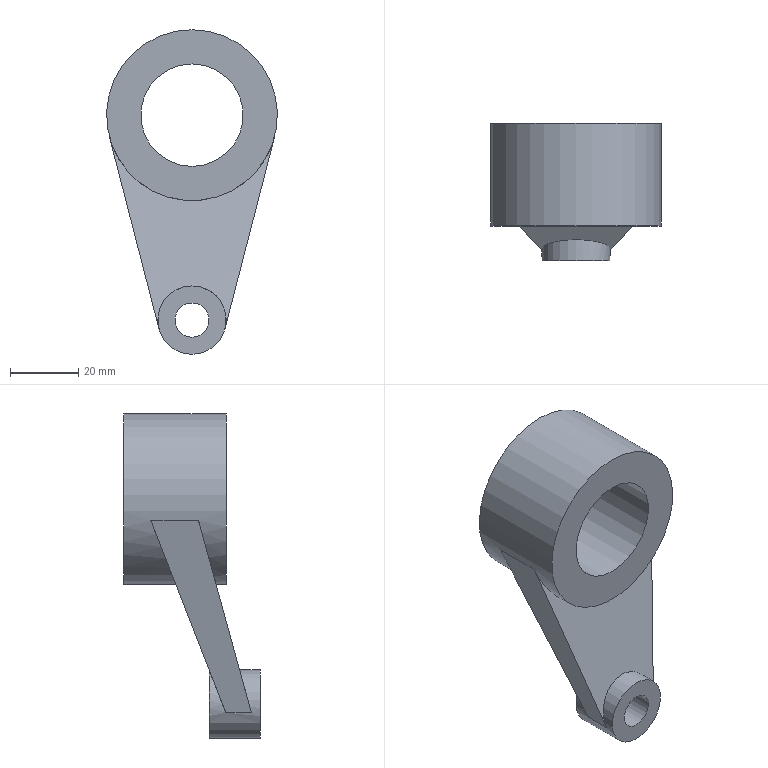Component | NX | WORKPIECE | 1 solid | 12 faces | box 50 x 40 x 95 mm | volume 52074 mm3 | plane 8 | cylinder 4 | commonest cylinder face diameters 50 x1 30 x1 20 x1 10 x1
STEP:
#1=CARTESIAN_POINT('',(0.,0.,0.));
#2=DIRECTION('',(0.,0.,1.));
#3=DIRECTION('',(1.,0.,0.));
#4=AXIS2_PLACEMENT_3D('',#1,#2,#3);
#5=CARTESIAN_POINT('',(-38.364,45.603,0.0009287));
#6=VERTEX_POINT('',#5);
#7=CARTESIAN_POINT('',(-28.68,50.48,12.5));
#8=VERTEX_POINT('',#7);
#9=CARTESIAN_POINT('',(-28.681,46.579,2.5));
#10=DIRECTION('',(-0.00003485,0.9316,-0.3634));
#11=DIRECTION('',(-0.00008933,-0.3634,-0.9316));
#12=AXIS2_PLACEMENT_3D('',#9,#10,#11);
#13=ELLIPSE('',#12,10.734,10.);
#14=CARTESIAN_POINT('',(1.318,43.947,-4.249));
#15=DIRECTION('',(0.00003485,-0.9316,0.3634));
#16=DIRECTION('',(-0.00008933,-0.3634,-0.9316));
#17=AXIS2_PLACEMENT_3D('',#14,#15,#16);
#18=PLANE('',#17);
#19=CARTESIAN_POINT('',(3.492,-30.));
#20=CARTESIAN_POINT('',(3.492,-47.321));
#21=CARTESIAN_POINT('',(-12.609,-38.66));
#22=CARTESIAN_POINT('',(-28.71,-30.));
#23=CARTESIAN_POINT('',(-12.609,-21.34));
#24=CARTESIAN_POINT('',(3.492,-12.679));
#25=CARTESIAN_POINT('',(3.492,-30.));
#26=(BOUNDED_CURVE()B_SPLINE_CURVE(2,(#19,#20,#21,#22,#23,#24,#25),.UNSPECIFIED.,.T.,.F.)B_SPLINE_CURVE_WITH_KNOTS((1,2,2,2,2,1),(-2.094,0.,2.094,4.189,6.283,8.378),.UNSPECIFIED.)CURVE()GEOMETRIC_REPRESENTATION_ITEM()RATIONAL_B_SPLINE_CURVE((1.,0.5,1.,0.5,1.,0.5,1.))REPRESENTATION_ITEM(''));
#27=(GEOMETRIC_REPRESENTATION_CONTEXT(2)PARAMETRIC_REPRESENTATION_CONTEXT()REPRESENTATION_CONTEXT('',''));
#28=DEFINITIONAL_REPRESENTATION('',(#26),#27);
#29=PCURVE('',#18,#28);
#30=CARTESIAN_POINT('',(-28.681,50.5,2.5));
#31=DIRECTION('',(0.,-1.,0.));
#32=DIRECTION('',(-0.00009588,0.,-1.));
#33=AXIS2_PLACEMENT_3D('',#30,#31,#32);
#34=CYLINDRICAL_SURFACE('',#33,10.);
#35=CARTESIAN_POINT('',(4.965,4.897));
#36=CARTESIAN_POINT('',(4.91,4.688));
#37=CARTESIAN_POINT('',(4.799,4.261));
#38=CARTESIAN_POINT('',(4.634,3.613));
#39=CARTESIAN_POINT('',(4.468,2.972));
#40=CARTESIAN_POINT('',(4.302,2.358));
#41=CARTESIAN_POINT('',(4.136,1.786));
#42=CARTESIAN_POINT('',(3.97,1.273));
#43=CARTESIAN_POINT('',(3.805,0.8326));
#44=CARTESIAN_POINT('',(3.639,0.4769));
#45=CARTESIAN_POINT('',(3.473,0.2156));
#46=CARTESIAN_POINT('',(3.307,0.05589));
#47=CARTESIAN_POINT('',(3.142,0.002165));
#48=CARTESIAN_POINT('',(2.976,0.05589));
#49=CARTESIAN_POINT('',(2.81,0.2156));
#50=CARTESIAN_POINT('',(2.644,0.4769));
#51=CARTESIAN_POINT('',(2.479,0.8326));
#52=CARTESIAN_POINT('',(2.313,1.273));
#53=CARTESIAN_POINT('',(2.147,1.786));
#54=CARTESIAN_POINT('',(1.981,2.358));
#55=CARTESIAN_POINT('',(1.815,2.972));
#56=CARTESIAN_POINT('',(1.65,3.613));
#57=CARTESIAN_POINT('',(1.484,4.261));
#58=CARTESIAN_POINT('',(1.373,4.688));
#59=CARTESIAN_POINT('',(1.318,4.897));
#60=B_SPLINE_CURVE_WITH_KNOTS('',3,(#35,#36,#37,#38,#39,#40,#41,#42,#43,#44,#45,#46,#47,#48,#49,#50,#51,#52,#53,#54,#55,#56,#57,#58,#59),.UNSPECIFIED.,.F.,.F.,(4,1,1,1,1,1,1,1,1,1,1,1,1,1,1,1,1,1,1,1,1,1,4),(1.318,1.484,1.65,1.815,1.981,2.147,2.313,2.479,2.644,2.81,2.976,3.142,3.307,3.473,3.639,3.805,3.97,4.136,4.302,4.468,4.634,4.799,4.965),.QUASI_UNIFORM_KNOTS.);
#61=(GEOMETRIC_REPRESENTATION_CONTEXT(2)PARAMETRIC_REPRESENTATION_CONTEXT()REPRESENTATION_CONTEXT('',''));
#62=DEFINITIONAL_REPRESENTATION('',(#60),#61);
#63=PCURVE('',#34,#62);
#64=SURFACE_CURVE('',#13,(#29,#63),.PCURVE_S1.);
#65=EDGE_CURVE('',#6,#8,#64,.T.);
#66=ORIENTED_EDGE('',*,*,#65,.F.);
#67=CARTESIAN_POINT('',(-52.882,67.548,56.252));
#68=VERTEX_POINT('',#67);
#69=CARTESIAN_POINT('',(-35.158,40.758,-12.42));
#70=DIRECTION('',(-0.2338,0.3534,0.9058));
#71=VECTOR('',#70,1.);
#72=LINE('',#69,#71);
#73=CARTESIAN_POINT('',(8.774,-36.475));
#74=DIRECTION('',(-0.9723,-0.2339));
#75=VECTOR('',#74,1.);
#76=LINE('',#73,#75);
#77=(GEOMETRIC_REPRESENTATION_CONTEXT(2)PARAMETRIC_REPRESENTATION_CONTEXT()REPRESENTATION_CONTEXT('',''));
#78=DEFINITIONAL_REPRESENTATION('',(#76),#77);
#79=PCURVE('',#18,#78);
#80=CARTESIAN_POINT('',(-64.414,-24.5,100.934));
#81=DIRECTION('',(0.9683,0.,0.2499));
#82=DIRECTION('',(0.2499,0.,-0.9683));
#83=AXIS2_PLACEMENT_3D('',#80,#81,#82);
#84=PLANE('',#83);
#85=CARTESIAN_POINT('',(117.069,65.258));
#86=DIRECTION('',(-0.9355,0.3534));
#87=VECTOR('',#86,1.);
#88=LINE('',#85,#87);
#89=(GEOMETRIC_REPRESENTATION_CONTEXT(2)PARAMETRIC_REPRESENTATION_CONTEXT()REPRESENTATION_CONTEXT('',''));
#90=DEFINITIONAL_REPRESENTATION('',(#88),#89);
#91=PCURVE('',#84,#90);
#92=SURFACE_CURVE('',#72,(#79,#91),.PCURVE_S1.);
#93=EDGE_CURVE('',#6,#68,#92,.T.);
#94=ORIENTED_EDGE('',*,*,#93,.T.);
#95=CARTESIAN_POINT('',(-4.47,67.548,56.248));
#96=VERTEX_POINT('',#95);
#97=CARTESIAN_POINT('',(-28.675,69.986,62.5));
#98=DIRECTION('',(0.00003485,-0.9316,0.3634));
#99=DIRECTION('',(-0.00008933,-0.3634,-0.9316));
#100=AXIS2_PLACEMENT_3D('',#97,#98,#99);
#101=ELLIPSE('',#100,26.835,25.);
#102=CARTESIAN_POINT('',(-71.646,-30.));
#103=DIRECTION('',(1.,-0.));
#104=AXIS2_PLACEMENT_2D('',#102,#103);
#105=ELLIPSE('',#104,26.835,25.);
#106=(GEOMETRIC_REPRESENTATION_CONTEXT(2)PARAMETRIC_REPRESENTATION_CONTEXT()REPRESENTATION_CONTEXT('',''));
#107=DEFINITIONAL_REPRESENTATION('',(#105),#106);
#108=PCURVE('',#18,#107);
#109=CARTESIAN_POINT('',(-28.675,75.5,62.5));
#110=DIRECTION('',(0.,-1.,0.));
#111=DIRECTION('',(-0.00009588,0.,-1.));
#112=AXIS2_PLACEMENT_3D('',#109,#110,#111);
#113=CYLINDRICAL_SURFACE('',#112,25.);
#114=CARTESIAN_POINT('',(4.965,7.952));
#115=CARTESIAN_POINT('',(5.005,8.329));
#116=CARTESIAN_POINT('',(5.085,9.072));
#117=CARTESIAN_POINT('',(5.205,10.135));
#118=CARTESIAN_POINT('',(5.325,11.132));
#119=CARTESIAN_POINT('',(5.444,12.048));
#120=CARTESIAN_POINT('',(5.564,12.871));
#121=CARTESIAN_POINT('',(5.684,13.588));
#122=CARTESIAN_POINT('',(5.804,14.189));
#123=CARTESIAN_POINT('',(5.924,14.665));
#124=CARTESIAN_POINT('',(6.044,15.011));
#125=CARTESIAN_POINT('',(6.163,15.22));
#126=CARTESIAN_POINT('',(6.283,15.29));
#127=CARTESIAN_POINT('',(6.403,15.22));
#128=CARTESIAN_POINT('',(6.523,15.011));
#129=CARTESIAN_POINT('',(6.643,14.665));
#130=CARTESIAN_POINT('',(6.763,14.189));
#131=CARTESIAN_POINT('',(6.882,13.588));
#132=CARTESIAN_POINT('',(7.002,12.871));
#133=CARTESIAN_POINT('',(7.122,12.048));
#134=CARTESIAN_POINT('',(7.242,11.132));
#135=CARTESIAN_POINT('',(7.362,10.135));
#136=CARTESIAN_POINT('',(7.481,9.072));
#137=CARTESIAN_POINT('',(7.561,8.329));
#138=CARTESIAN_POINT('',(7.601,7.952));
#139=B_SPLINE_CURVE_WITH_KNOTS('',3,(#114,#115,#116,#117,#118,#119,#120,#121,#122,#123,#124,#125,#126,#127,#128,#129,#130,#131,#132,#133,#134,#135,#136,#137,#138),.UNSPECIFIED.,.F.,.F.,(4,1,1,1,1,1,1,1,1,1,1,1,1,1,1,1,1,1,1,1,1,1,4),(4.965,5.085,5.205,5.325,5.444,5.564,5.684,5.804,5.924,6.044,6.163,6.283,6.403,6.523,6.643,6.763,6.882,7.002,7.122,7.242,7.362,7.481,7.601),.QUASI_UNIFORM_KNOTS.);
#140=(GEOMETRIC_REPRESENTATION_CONTEXT(2)PARAMETRIC_REPRESENTATION_CONTEXT()REPRESENTATION_CONTEXT('',''));
#141=DEFINITIONAL_REPRESENTATION('',(#139),#140);
#142=PCURVE('',#113,#141);
#143=SURFACE_CURVE('',#101,(#108,#142),.PCURVE_S1.);
#144=EDGE_CURVE('',#68,#96,#143,.T.);
#145=ORIENTED_EDGE('',*,*,#144,.T.);
#146=CARTESIAN_POINT('',(-18.999,45.603,-0.0009281));
#147=VERTEX_POINT('',#146);
#148=CARTESIAN_POINT('',(-24.794,36.85,-22.438));
#149=DIRECTION('',(0.234,0.3534,0.9058));
#150=VECTOR('',#149,1.);
#151=LINE('',#148,#150);
#152=CARTESIAN_POINT('',(19.527,-26.111));
#153=DIRECTION('',(-0.9723,0.2339));
#154=VECTOR('',#153,1.);
#155=LINE('',#152,#154);
#156=(GEOMETRIC_REPRESENTATION_CONTEXT(2)PARAMETRIC_REPRESENTATION_CONTEXT()REPRESENTATION_CONTEXT('',''));
#157=DEFINITIONAL_REPRESENTATION('',(#155),#156);
#158=PCURVE('',#18,#157);
#159=CARTESIAN_POINT('',(-18.999,-24.5,-0.0009281));
#160=DIRECTION('',(-0.9682,0.,0.2501));
#161=DIRECTION('',(0.2501,0.,0.9682));
#162=AXIS2_PLACEMENT_3D('',#159,#160,#161);
#163=PLANE('',#162);
#164=CARTESIAN_POINT('',(-23.174,61.35));
#165=DIRECTION('',(0.9355,0.3534));
#166=VECTOR('',#165,1.);
#167=LINE('',#164,#166);
#168=(GEOMETRIC_REPRESENTATION_CONTEXT(2)PARAMETRIC_REPRESENTATION_CONTEXT()REPRESENTATION_CONTEXT('',''));
#169=DEFINITIONAL_REPRESENTATION('',(#167),#168);
#170=PCURVE('',#163,#169);
#171=SURFACE_CURVE('',#151,(#158,#170),.PCURVE_S1.);
#172=EDGE_CURVE('',#147,#96,#171,.T.);
#173=ORIENTED_EDGE('',*,*,#172,.F.);
#174=CARTESIAN_POINT('',(-28.681,46.579,2.5));
#175=DIRECTION('',(-0.00003485,0.9316,-0.3634));
#176=DIRECTION('',(-0.00008933,-0.3634,-0.9316));
#177=AXIS2_PLACEMENT_3D('',#174,#175,#176);
#178=ELLIPSE('',#177,10.734,10.);
#179=CARTESIAN_POINT('',(3.492,-30.));
#180=CARTESIAN_POINT('',(3.492,-47.321));
#181=CARTESIAN_POINT('',(-12.609,-38.66));
#182=CARTESIAN_POINT('',(-28.71,-30.));
#183=CARTESIAN_POINT('',(-12.609,-21.34));
#184=CARTESIAN_POINT('',(3.492,-12.679));
#185=CARTESIAN_POINT('',(3.492,-30.));
#186=(BOUNDED_CURVE()B_SPLINE_CURVE(2,(#179,#180,#181,#182,#183,#184,#185),.UNSPECIFIED.,.T.,.F.)B_SPLINE_CURVE_WITH_KNOTS((1,2,2,2,2,1),(-2.094,0.,2.094,4.189,6.283,8.378),.UNSPECIFIED.)CURVE()GEOMETRIC_REPRESENTATION_ITEM()RATIONAL_B_SPLINE_CURVE((1.,0.5,1.,0.5,1.,0.5,1.))REPRESENTATION_ITEM(''));
#187=(GEOMETRIC_REPRESENTATION_CONTEXT(2)PARAMETRIC_REPRESENTATION_CONTEXT()REPRESENTATION_CONTEXT('',''));
#188=DEFINITIONAL_REPRESENTATION('',(#186),#187);
#189=PCURVE('',#18,#188);
#190=CARTESIAN_POINT('',(11.248,4.897));
#191=CARTESIAN_POINT('',(11.193,4.688));
#192=CARTESIAN_POINT('',(11.082,4.261));
#193=CARTESIAN_POINT('',(10.917,3.613));
#194=CARTESIAN_POINT('',(10.751,2.972));
#195=CARTESIAN_POINT('',(10.585,2.358));
#196=CARTESIAN_POINT('',(10.419,1.786));
#197=CARTESIAN_POINT('',(10.254,1.273));
#198=CARTESIAN_POINT('',(10.088,0.8326));
#199=CARTESIAN_POINT('',(9.922,0.4769));
#200=CARTESIAN_POINT('',(9.756,0.2156));
#201=CARTESIAN_POINT('',(9.591,0.05589));
#202=CARTESIAN_POINT('',(9.425,0.002165));
#203=CARTESIAN_POINT('',(9.259,0.05589));
#204=CARTESIAN_POINT('',(9.093,0.2156));
#205=CARTESIAN_POINT('',(8.927,0.4769));
#206=CARTESIAN_POINT('',(8.762,0.8326));
#207=CARTESIAN_POINT('',(8.596,1.273));
#208=CARTESIAN_POINT('',(8.43,1.786));
#209=CARTESIAN_POINT('',(8.264,2.358));
#210=CARTESIAN_POINT('',(8.099,2.972));
#211=CARTESIAN_POINT('',(7.933,3.613));
#212=CARTESIAN_POINT('',(7.767,4.261));
#213=CARTESIAN_POINT('',(7.657,4.688));
#214=CARTESIAN_POINT('',(7.601,4.897));
#215=B_SPLINE_CURVE_WITH_KNOTS('',3,(#190,#191,#192,#193,#194,#195,#196,#197,#198,#199,#200,#201,#202,#203,#204,#205,#206,#207,#208,#209,#210,#211,#212,#213,#214),.UNSPECIFIED.,.F.,.F.,(4,1,1,1,1,1,1,1,1,1,1,1,1,1,1,1,1,1,1,1,1,1,4),(1.318,1.484,1.65,1.815,1.981,2.147,2.313,2.479,2.644,2.81,2.976,3.142,3.307,3.473,3.639,3.805,3.97,4.136,4.302,4.468,4.634,4.799,4.965),.QUASI_UNIFORM_KNOTS.);
#216=(GEOMETRIC_REPRESENTATION_CONTEXT(2)PARAMETRIC_REPRESENTATION_CONTEXT()REPRESENTATION_CONTEXT('',''));
#217=DEFINITIONAL_REPRESENTATION('',(#215),#216);
#218=PCURVE('',#34,#217);
#219=SURFACE_CURVE('',#178,(#189,#218),.PCURVE_S1.);
#220=EDGE_CURVE('',#8,#147,#219,.T.);
#221=ORIENTED_EDGE('',*,*,#220,.F.);
#222=EDGE_LOOP('',(#66,#94,#145,#173,#221));
#223=FACE_BOUND('',#222,.T.);
#224=ADVANCED_FACE('',(#223),#18,.F.);
#225=CARTESIAN_POINT('',(-18.999,38.133,-0.0009281));
#226=VERTEX_POINT('',#225);
#227=CARTESIAN_POINT('',(-28.68,41.574,12.5));
#228=VERTEX_POINT('',#227);
#229=CARTESIAN_POINT('',(-28.681,38.821,2.5));
#230=DIRECTION('',(0.00002545,-0.9641,0.2654));
#231=DIRECTION('',(-0.00009245,-0.2654,-0.9641));
#232=AXIS2_PLACEMENT_3D('',#229,#230,#231);
#233=ELLIPSE('',#232,10.372,10.);
#234=CARTESIAN_POINT('',(1.326,58.322,73.338));
#235=DIRECTION('',(-0.00002545,0.9641,-0.2654));
#236=DIRECTION('',(0.00009245,0.2654,0.9641));
#237=AXIS2_PLACEMENT_3D('',#234,#235,#236);
#238=PLANE('',#237);
#239=CARTESIAN_POINT('',(-83.848,-30.));
#240=CARTESIAN_POINT('',(-83.848,-12.679));
#241=CARTESIAN_POINT('',(-68.29,-21.34));
#242=CARTESIAN_POINT('',(-52.732,-30.));
#243=CARTESIAN_POINT('',(-68.29,-38.66));
#244=CARTESIAN_POINT('',(-83.848,-47.321));
#245=CARTESIAN_POINT('',(-83.848,-30.));
#246=(BOUNDED_CURVE()B_SPLINE_CURVE(2,(#239,#240,#241,#242,#243,#244,#245),.UNSPECIFIED.,.T.,.F.)B_SPLINE_CURVE_WITH_KNOTS((1,2,2,2,2,1),(-2.094,0.,2.094,4.189,6.283,8.378),.UNSPECIFIED.)CURVE()GEOMETRIC_REPRESENTATION_ITEM()RATIONAL_B_SPLINE_CURVE((1.,0.5,1.,0.5,1.,0.5,1.))REPRESENTATION_ITEM(''));
#247=(GEOMETRIC_REPRESENTATION_CONTEXT(2)PARAMETRIC_REPRESENTATION_CONTEXT()REPRESENTATION_CONTEXT('',''));
#248=DEFINITIONAL_REPRESENTATION('',(#246),#247);
#249=PCURVE('',#238,#248);
#250=CARTESIAN_POINT('',(7.601,12.367));
#251=CARTESIAN_POINT('',(7.657,12.22));
#252=CARTESIAN_POINT('',(7.767,11.919));
#253=CARTESIAN_POINT('',(7.933,11.461));
#254=CARTESIAN_POINT('',(8.099,11.009));
#255=CARTESIAN_POINT('',(8.264,10.576));
#256=CARTESIAN_POINT('',(8.43,10.172));
#257=CARTESIAN_POINT('',(8.596,9.81));
#258=CARTESIAN_POINT('',(8.762,9.5));
#259=CARTESIAN_POINT('',(8.927,9.249));
#260=CARTESIAN_POINT('',(9.093,9.064));
#261=CARTESIAN_POINT('',(9.259,8.952));
#262=CARTESIAN_POINT('',(9.425,8.914));
#263=CARTESIAN_POINT('',(9.591,8.952));
#264=CARTESIAN_POINT('',(9.756,9.064));
#265=CARTESIAN_POINT('',(9.922,9.249));
#266=CARTESIAN_POINT('',(10.088,9.5));
#267=CARTESIAN_POINT('',(10.254,9.81));
#268=CARTESIAN_POINT('',(10.419,10.172));
#269=CARTESIAN_POINT('',(10.585,10.576));
#270=CARTESIAN_POINT('',(10.751,11.009));
#271=CARTESIAN_POINT('',(10.917,11.461));
#272=CARTESIAN_POINT('',(11.082,11.919));
#273=CARTESIAN_POINT('',(11.193,12.22));
#274=CARTESIAN_POINT('',(11.248,12.367));
#275=B_SPLINE_CURVE_WITH_KNOTS('',3,(#250,#251,#252,#253,#254,#255,#256,#257,#258,#259,#260,#261,#262,#263,#264,#265,#266,#267,#268,#269,#270,#271,#272,#273,#274),.UNSPECIFIED.,.F.,.F.,(4,1,1,1,1,1,1,1,1,1,1,1,1,1,1,1,1,1,1,1,1,1,4),(1.318,1.484,1.65,1.815,1.981,2.147,2.313,2.479,2.644,2.81,2.976,3.142,3.307,3.473,3.639,3.805,3.97,4.136,4.302,4.468,4.634,4.799,4.965),.QUASI_UNIFORM_KNOTS.);
#276=(GEOMETRIC_REPRESENTATION_CONTEXT(2)PARAMETRIC_REPRESENTATION_CONTEXT()REPRESENTATION_CONTEXT('',''));
#277=DEFINITIONAL_REPRESENTATION('',(#275),#276);
#278=PCURVE('',#34,#277);
#279=SURFACE_CURVE('',#233,(#249,#278),.PCURVE_S1.);
#280=EDGE_CURVE('',#226,#228,#279,.T.);
#281=ORIENTED_EDGE('',*,*,#280,.F.);
#282=CARTESIAN_POINT('',(-4.47,53.617,56.248));
#283=VERTEX_POINT('',#282);
#284=CARTESIAN_POINT('',(-22.897,33.978,-15.092));
#285=DIRECTION('',(-0.2417,-0.2575,-0.9356));
#286=VECTOR('',#285,1.);
#287=LINE('',#284,#286);
#288=CARTESIAN_POINT('',(-91.722,-24.214));
#289=DIRECTION('',(-0.9704,-0.2416));
#290=VECTOR('',#289,1.);
#291=LINE('',#288,#290);
#292=(GEOMETRIC_REPRESENTATION_CONTEXT(2)PARAMETRIC_REPRESENTATION_CONTEXT()REPRESENTATION_CONTEXT('',''));
#293=DEFINITIONAL_REPRESENTATION('',(#291),#292);
#294=PCURVE('',#238,#293);
#295=CARTESIAN_POINT('',(-15.586,58.478));
#296=DIRECTION('',(-0.9663,-0.2575));
#297=VECTOR('',#296,1.);
#298=LINE('',#295,#297);
#299=(GEOMETRIC_REPRESENTATION_CONTEXT(2)PARAMETRIC_REPRESENTATION_CONTEXT()REPRESENTATION_CONTEXT('',''));
#300=DEFINITIONAL_REPRESENTATION('',(#298),#299);
#301=PCURVE('',#163,#300);
#302=SURFACE_CURVE('',#287,(#294,#301),.PCURVE_S1.);
#303=EDGE_CURVE('',#283,#226,#302,.T.);
#304=ORIENTED_EDGE('',*,*,#303,.F.);
#305=CARTESIAN_POINT('',(-52.882,53.617,56.252));
#306=VERTEX_POINT('',#305);
#307=CARTESIAN_POINT('',(-28.675,55.337,62.5));
#308=DIRECTION('',(-0.00002545,0.9641,-0.2654));
#309=DIRECTION('',(-0.00009245,-0.2654,-0.9641));
#310=AXIS2_PLACEMENT_3D('',#307,#308,#309);
#311=ELLIPSE('',#310,25.93,25.);
#312=CARTESIAN_POINT('',(-11.245,-30.));
#313=DIRECTION('',(-1.,-0.));
#314=AXIS2_PLACEMENT_2D('',#312,#313);
#315=ELLIPSE('',#314,25.93,25.);
#316=(GEOMETRIC_REPRESENTATION_CONTEXT(2)PARAMETRIC_REPRESENTATION_CONTEXT()REPRESENTATION_CONTEXT('',''));
#317=DEFINITIONAL_REPRESENTATION('',(#315),#316);
#318=PCURVE('',#238,#317);
#319=CARTESIAN_POINT('',(7.601,21.883));
#320=CARTESIAN_POINT('',(7.561,22.149));
#321=CARTESIAN_POINT('',(7.481,22.673));
#322=CARTESIAN_POINT('',(7.362,23.423));
#323=CARTESIAN_POINT('',(7.242,24.127));
#324=CARTESIAN_POINT('',(7.122,24.773));
#325=CARTESIAN_POINT('',(7.002,25.354));
#326=CARTESIAN_POINT('',(6.882,25.859));
#327=CARTESIAN_POINT('',(6.763,26.284));
#328=CARTESIAN_POINT('',(6.643,26.62));
#329=CARTESIAN_POINT('',(6.523,26.864));
#330=CARTESIAN_POINT('',(6.403,27.012));
#331=CARTESIAN_POINT('',(6.283,27.061));
#332=CARTESIAN_POINT('',(6.163,27.012));
#333=CARTESIAN_POINT('',(6.044,26.864));
#334=CARTESIAN_POINT('',(5.924,26.62));
#335=CARTESIAN_POINT('',(5.804,26.284));
#336=CARTESIAN_POINT('',(5.684,25.859));
#337=CARTESIAN_POINT('',(5.564,25.354));
#338=CARTESIAN_POINT('',(5.444,24.773));
#339=CARTESIAN_POINT('',(5.325,24.127));
#340=CARTESIAN_POINT('',(5.205,23.423));
#341=CARTESIAN_POINT('',(5.085,22.673));
#342=CARTESIAN_POINT('',(5.005,22.149));
#343=CARTESIAN_POINT('',(4.965,21.883));
#344=B_SPLINE_CURVE_WITH_KNOTS('',3,(#319,#320,#321,#322,#323,#324,#325,#326,#327,#328,#329,#330,#331,#332,#333,#334,#335,#336,#337,#338,#339,#340,#341,#342,#343),.UNSPECIFIED.,.F.,.F.,(4,1,1,1,1,1,1,1,1,1,1,1,1,1,1,1,1,1,1,1,1,1,4),(4.965,5.085,5.205,5.325,5.444,5.564,5.684,5.804,5.924,6.044,6.163,6.283,6.403,6.523,6.643,6.763,6.882,7.002,7.122,7.242,7.362,7.481,7.601),.QUASI_UNIFORM_KNOTS.);
#345=(GEOMETRIC_REPRESENTATION_CONTEXT(2)PARAMETRIC_REPRESENTATION_CONTEXT()REPRESENTATION_CONTEXT('',''));
#346=DEFINITIONAL_REPRESENTATION('',(#344),#345);
#347=PCURVE('',#113,#346);
#348=SURFACE_CURVE('',#311,(#318,#347),.PCURVE_S1.);
#349=EDGE_CURVE('',#283,#306,#348,.T.);
#350=ORIENTED_EDGE('',*,*,#349,.T.);
#351=CARTESIAN_POINT('',(-38.364,38.133,0.0009287));
#352=VERTEX_POINT('',#351);
#353=CARTESIAN_POINT('',(-53.874,54.675,60.096));
#354=DIRECTION('',(0.2415,-0.2575,-0.9356));
#355=VECTOR('',#354,1.);
#356=LINE('',#353,#355);
#357=CARTESIAN_POINT('',(-13.741,-55.198));
#358=DIRECTION('',(-0.9704,0.2416));
#359=VECTOR('',#358,1.);
#360=LINE('',#357,#359);
#361=(GEOMETRIC_REPRESENTATION_CONTEXT(2)PARAMETRIC_REPRESENTATION_CONTEXT()REPRESENTATION_CONTEXT('',''));
#362=DEFINITIONAL_REPRESENTATION('',(#360),#361);
#363=PCURVE('',#238,#362);
#364=CARTESIAN_POINT('',(42.177,79.175));
#365=DIRECTION('',(0.9663,-0.2575));
#366=VECTOR('',#365,1.);
#367=LINE('',#364,#366);
#368=(GEOMETRIC_REPRESENTATION_CONTEXT(2)PARAMETRIC_REPRESENTATION_CONTEXT()REPRESENTATION_CONTEXT('',''));
#369=DEFINITIONAL_REPRESENTATION('',(#367),#368);
#370=PCURVE('',#84,#369);
#371=SURFACE_CURVE('',#356,(#363,#370),.PCURVE_S1.);
#372=EDGE_CURVE('',#306,#352,#371,.T.);
#373=ORIENTED_EDGE('',*,*,#372,.T.);
#374=CARTESIAN_POINT('',(-28.681,38.821,2.5));
#375=DIRECTION('',(0.00002545,-0.9641,0.2654));
#376=DIRECTION('',(-0.00009245,-0.2654,-0.9641));
#377=AXIS2_PLACEMENT_3D('',#374,#375,#376);
#378=ELLIPSE('',#377,10.372,10.);
#379=CARTESIAN_POINT('',(-83.848,-30.));
#380=CARTESIAN_POINT('',(-83.848,-12.679));
#381=CARTESIAN_POINT('',(-68.29,-21.34));
#382=CARTESIAN_POINT('',(-52.732,-30.));
#383=CARTESIAN_POINT('',(-68.29,-38.66));
#384=CARTESIAN_POINT('',(-83.848,-47.321));
#385=CARTESIAN_POINT('',(-83.848,-30.));
#386=(BOUNDED_CURVE()B_SPLINE_CURVE(2,(#379,#380,#381,#382,#383,#384,#385),.UNSPECIFIED.,.T.,.F.)B_SPLINE_CURVE_WITH_KNOTS((1,2,2,2,2,1),(-2.094,0.,2.094,4.189,6.283,8.378),.UNSPECIFIED.)CURVE()GEOMETRIC_REPRESENTATION_ITEM()RATIONAL_B_SPLINE_CURVE((1.,0.5,1.,0.5,1.,0.5,1.))REPRESENTATION_ITEM(''));
#387=(GEOMETRIC_REPRESENTATION_CONTEXT(2)PARAMETRIC_REPRESENTATION_CONTEXT()REPRESENTATION_CONTEXT('',''));
#388=DEFINITIONAL_REPRESENTATION('',(#386),#387);
#389=PCURVE('',#238,#388);
#390=CARTESIAN_POINT('',(1.318,12.367));
#391=CARTESIAN_POINT('',(1.373,12.22));
#392=CARTESIAN_POINT('',(1.484,11.919));
#393=CARTESIAN_POINT('',(1.65,11.461));
#394=CARTESIAN_POINT('',(1.815,11.009));
#395=CARTESIAN_POINT('',(1.981,10.576));
#396=CARTESIAN_POINT('',(2.147,10.172));
#397=CARTESIAN_POINT('',(2.313,9.81));
#398=CARTESIAN_POINT('',(2.479,9.5));
#399=CARTESIAN_POINT('',(2.644,9.249));
#400=CARTESIAN_POINT('',(2.81,9.064));
#401=CARTESIAN_POINT('',(2.976,8.952));
#402=CARTESIAN_POINT('',(3.142,8.914));
#403=CARTESIAN_POINT('',(3.307,8.952));
#404=CARTESIAN_POINT('',(3.473,9.064));
#405=CARTESIAN_POINT('',(3.639,9.249));
#406=CARTESIAN_POINT('',(3.805,9.5));
#407=CARTESIAN_POINT('',(3.97,9.81));
#408=CARTESIAN_POINT('',(4.136,10.172));
#409=CARTESIAN_POINT('',(4.302,10.576));
#410=CARTESIAN_POINT('',(4.468,11.009));
#411=CARTESIAN_POINT('',(4.634,11.461));
#412=CARTESIAN_POINT('',(4.799,11.919));
#413=CARTESIAN_POINT('',(4.91,12.22));
#414=CARTESIAN_POINT('',(4.965,12.367));
#415=B_SPLINE_CURVE_WITH_KNOTS('',3,(#390,#391,#392,#393,#394,#395,#396,#397,#398,#399,#400,#401,#402,#403,#404,#405,#406,#407,#408,#409,#410,#411,#412,#413,#414),.UNSPECIFIED.,.F.,.F.,(4,1,1,1,1,1,1,1,1,1,1,1,1,1,1,1,1,1,1,1,1,1,4),(1.318,1.484,1.65,1.815,1.981,2.147,2.313,2.479,2.644,2.81,2.976,3.142,3.307,3.473,3.639,3.805,3.97,4.136,4.302,4.468,4.634,4.799,4.965),.QUASI_UNIFORM_KNOTS.);
#416=(GEOMETRIC_REPRESENTATION_CONTEXT(2)PARAMETRIC_REPRESENTATION_CONTEXT()REPRESENTATION_CONTEXT('',''));
#417=DEFINITIONAL_REPRESENTATION('',(#415),#416);
#418=PCURVE('',#34,#417);
#419=SURFACE_CURVE('',#378,(#389,#418),.PCURVE_S1.);
#420=EDGE_CURVE('',#228,#352,#419,.T.);
#421=ORIENTED_EDGE('',*,*,#420,.F.);
#422=EDGE_LOOP('',(#281,#304,#350,#373,#421));
#423=FACE_BOUND('',#422,.T.);
#424=ADVANCED_FACE('',(#423),#238,.F.);
#425=CARTESIAN_POINT('',(-28.673,45.5,87.5));
#426=VERTEX_POINT('',#425);
#427=CARTESIAN_POINT('',(-28.675,45.5,62.5));
#428=DIRECTION('',(0.,1.,0.));
#429=DIRECTION('',(0.00009588,0.,1.));
#430=AXIS2_PLACEMENT_3D('',#427,#428,#429);
#431=CIRCLE('',#430,25.);
#432=CARTESIAN_POINT('',(9.425,30.));
#433=DIRECTION('',(-1.,0.));
#434=VECTOR('',#433,1.);
#435=LINE('',#432,#434);
#436=(GEOMETRIC_REPRESENTATION_CONTEXT(2)PARAMETRIC_REPRESENTATION_CONTEXT()REPRESENTATION_CONTEXT('',''));
#437=DEFINITIONAL_REPRESENTATION('',(#435),#436);
#438=PCURVE('',#113,#437);
#439=CARTESIAN_POINT('',(-28.675,45.5,62.5));
#440=DIRECTION('',(0.,1.,0.));
#441=DIRECTION('',(0.00009588,0.,1.));
#442=AXIS2_PLACEMENT_3D('',#439,#440,#441);
#443=PLANE('',#442);
#444=CARTESIAN_POINT('',(0.,0.));
#445=DIRECTION('',(1.,0.));
#446=AXIS2_PLACEMENT_2D('',#444,#445);
#447=CIRCLE('',#446,25.);
#448=(GEOMETRIC_REPRESENTATION_CONTEXT(2)PARAMETRIC_REPRESENTATION_CONTEXT()REPRESENTATION_CONTEXT('',''));
#449=DEFINITIONAL_REPRESENTATION('',(#447),#448);
#450=PCURVE('',#443,#449);
#451=SURFACE_CURVE('',#431,(#438,#450),.PCURVE_S1.);
#452=EDGE_CURVE('',#426,#426,#451,.T.);
#453=ORIENTED_EDGE('',*,*,#452,.T.);
#454=CARTESIAN_POINT('',(-28.673,75.5,87.5));
#455=VERTEX_POINT('',#454);
#456=CARTESIAN_POINT('',(-28.673,75.5,87.5));
#457=CARTESIAN_POINT('',(-28.673,45.5,87.5));
#458=B_SPLINE_CURVE_WITH_KNOTS('',1,(#456,#457),.UNSPECIFIED.,.F.,.F.,(2,2),(0.,30.),.PIECEWISE_BEZIER_KNOTS.);
#459=CARTESIAN_POINT('',(3.142,0.));
#460=DIRECTION('',(0.,1.));
#461=VECTOR('',#460,1.);
#462=LINE('',#459,#461);
#463=(GEOMETRIC_REPRESENTATION_CONTEXT(2)PARAMETRIC_REPRESENTATION_CONTEXT()REPRESENTATION_CONTEXT('',''));
#464=DEFINITIONAL_REPRESENTATION('',(#462),#463);
#465=PCURVE('',#113,#464);
#466=CARTESIAN_POINT('',(9.425,0.));
#467=DIRECTION('',(0.,1.));
#468=VECTOR('',#467,1.);
#469=LINE('',#466,#468);
#470=(GEOMETRIC_REPRESENTATION_CONTEXT(2)PARAMETRIC_REPRESENTATION_CONTEXT()REPRESENTATION_CONTEXT('',''));
#471=DEFINITIONAL_REPRESENTATION('',(#469),#470);
#472=PCURVE('',#113,#471);
#473=SEAM_CURVE('',#458,(#465,#472),.PCURVE_S1.);
#474=EDGE_CURVE('',#455,#426,#473,.T.);
#475=ORIENTED_EDGE('',*,*,#474,.F.);
#476=CARTESIAN_POINT('',(-28.675,75.5,62.5));
#477=DIRECTION('',(0.,1.,0.));
#478=DIRECTION('',(0.00009588,0.,1.));
#479=AXIS2_PLACEMENT_3D('',#476,#477,#478);
#480=CIRCLE('',#479,25.);
#481=CARTESIAN_POINT('',(9.425,0.));
#482=DIRECTION('',(-1.,0.));
#483=VECTOR('',#482,1.);
#484=LINE('',#481,#483);
#485=(GEOMETRIC_REPRESENTATION_CONTEXT(2)PARAMETRIC_REPRESENTATION_CONTEXT()REPRESENTATION_CONTEXT('',''));
#486=DEFINITIONAL_REPRESENTATION('',(#484),#485);
#487=PCURVE('',#113,#486);
#488=CARTESIAN_POINT('',(-28.675,75.5,62.5));
#489=DIRECTION('',(0.,1.,0.));
#490=DIRECTION('',(0.00009588,0.,1.));
#491=AXIS2_PLACEMENT_3D('',#488,#489,#490);
#492=PLANE('',#491);
#493=CARTESIAN_POINT('',(0.,0.));
#494=DIRECTION('',(1.,0.));
#495=AXIS2_PLACEMENT_2D('',#493,#494);
#496=CIRCLE('',#495,25.);
#497=(GEOMETRIC_REPRESENTATION_CONTEXT(2)PARAMETRIC_REPRESENTATION_CONTEXT()REPRESENTATION_CONTEXT('',''));
#498=DEFINITIONAL_REPRESENTATION('',(#496),#497);
#499=PCURVE('',#492,#498);
#500=SURFACE_CURVE('',#480,(#487,#499),.PCURVE_S1.);
#501=EDGE_CURVE('',#455,#455,#500,.T.);
#502=ORIENTED_EDGE('',*,*,#501,.F.);
#503=ORIENTED_EDGE('',*,*,#474,.T.);
#504=EDGE_LOOP('',(#453,#475,#502,#503));
#505=FACE_BOUND('',#504,.T.);
#506=CARTESIAN_POINT('',(-4.47,66.269,56.248));
#507=DIRECTION('',(0.,-1.,0.));
#508=VECTOR('',#507,1.);
#509=LINE('',#506,#508);
#510=CARTESIAN_POINT('',(7.601,9.231));
#511=DIRECTION('',(0.,1.));
#512=VECTOR('',#511,1.);
#513=LINE('',#510,#512);
#514=(GEOMETRIC_REPRESENTATION_CONTEXT(2)PARAMETRIC_REPRESENTATION_CONTEXT()REPRESENTATION_CONTEXT('',''));
#515=DEFINITIONAL_REPRESENTATION('',(#513),#514);
#516=PCURVE('',#113,#515);
#517=CARTESIAN_POINT('',(58.095,90.769));
#518=DIRECTION('',(0.,-1.));
#519=VECTOR('',#518,1.);
#520=LINE('',#517,#519);
#521=(GEOMETRIC_REPRESENTATION_CONTEXT(2)PARAMETRIC_REPRESENTATION_CONTEXT()REPRESENTATION_CONTEXT('',''));
#522=DEFINITIONAL_REPRESENTATION('',(#520),#521);
#523=PCURVE('',#163,#522);
#524=SURFACE_CURVE('',#509,(#516,#523),.PCURVE_S1.);
#525=EDGE_CURVE('',#96,#283,#524,.T.);
#526=ORIENTED_EDGE('',*,*,#525,.F.);
#527=ORIENTED_EDGE('',*,*,#144,.F.);
#528=CARTESIAN_POINT('',(-52.882,66.269,56.252));
#529=DIRECTION('',(0.,-1.,0.));
#530=VECTOR('',#529,1.);
#531=LINE('',#528,#530);
#532=CARTESIAN_POINT('',(4.965,9.231));
#533=DIRECTION('',(0.,1.));
#534=VECTOR('',#533,1.);
#535=LINE('',#532,#534);
#536=(GEOMETRIC_REPRESENTATION_CONTEXT(2)PARAMETRIC_REPRESENTATION_CONTEXT()REPRESENTATION_CONTEXT('',''));
#537=DEFINITIONAL_REPRESENTATION('',(#535),#536);
#538=PCURVE('',#113,#537);
#539=CARTESIAN_POINT('',(46.146,90.769));
#540=DIRECTION('',(0.,-1.));
#541=VECTOR('',#540,1.);
#542=LINE('',#539,#541);
#543=(GEOMETRIC_REPRESENTATION_CONTEXT(2)PARAMETRIC_REPRESENTATION_CONTEXT()REPRESENTATION_CONTEXT('',''));
#544=DEFINITIONAL_REPRESENTATION('',(#542),#543);
#545=PCURVE('',#84,#544);
#546=SURFACE_CURVE('',#531,(#538,#545),.PCURVE_S1.);
#547=EDGE_CURVE('',#68,#306,#546,.T.);
#548=ORIENTED_EDGE('',*,*,#547,.T.);
#549=ORIENTED_EDGE('',*,*,#349,.F.);
#550=EDGE_LOOP('',(#526,#527,#548,#549));
#551=FACE_BOUND('',#550,.T.);
#552=ADVANCED_FACE('',(#505,#551),#113,.T.);
#553=CARTESIAN_POINT('',(-28.674,75.5,77.5));
#554=VERTEX_POINT('',#553);
#555=CARTESIAN_POINT('',(-28.675,75.5,62.5));
#556=DIRECTION('',(0.,1.,0.));
#557=DIRECTION('',(0.00009588,0.,1.));
#558=AXIS2_PLACEMENT_3D('',#555,#556,#557);
#559=CIRCLE('',#558,15.);
#560=CARTESIAN_POINT('',(-28.675,75.5,62.5));
#561=DIRECTION('',(0.,-1.,0.));
#562=DIRECTION('',(-0.00009588,0.,-1.));
#563=AXIS2_PLACEMENT_3D('',#560,#561,#562);
#564=CYLINDRICAL_SURFACE('',#563,15.);
#565=CARTESIAN_POINT('',(9.425,0.));
#566=DIRECTION('',(-1.,0.));
#567=VECTOR('',#566,1.);
#568=LINE('',#565,#567);
#569=(GEOMETRIC_REPRESENTATION_CONTEXT(2)PARAMETRIC_REPRESENTATION_CONTEXT()REPRESENTATION_CONTEXT('',''));
#570=DEFINITIONAL_REPRESENTATION('',(#568),#569);
#571=PCURVE('',#564,#570);
#572=CARTESIAN_POINT('',(0.,0.));
#573=DIRECTION('',(1.,0.));
#574=AXIS2_PLACEMENT_2D('',#572,#573);
#575=CIRCLE('',#574,15.);
#576=(GEOMETRIC_REPRESENTATION_CONTEXT(2)PARAMETRIC_REPRESENTATION_CONTEXT()REPRESENTATION_CONTEXT('',''));
#577=DEFINITIONAL_REPRESENTATION('',(#575),#576);
#578=PCURVE('',#492,#577);
#579=SURFACE_CURVE('',#559,(#571,#578),.PCURVE_S1.);
#580=EDGE_CURVE('',#554,#554,#579,.T.);
#581=ORIENTED_EDGE('',*,*,#580,.F.);
#582=CARTESIAN_POINT('',(-28.674,45.5,77.5));
#583=VERTEX_POINT('',#582);
#584=CARTESIAN_POINT('',(-28.674,75.5,77.5));
#585=CARTESIAN_POINT('',(-28.674,45.5,77.5));
#586=B_SPLINE_CURVE_WITH_KNOTS('',1,(#584,#585),.UNSPECIFIED.,.F.,.F.,(2,2),(0.,30.),.PIECEWISE_BEZIER_KNOTS.);
#587=CARTESIAN_POINT('',(9.425,0.));
#588=DIRECTION('',(0.,1.));
#589=VECTOR('',#588,1.);
#590=LINE('',#587,#589);
#591=(GEOMETRIC_REPRESENTATION_CONTEXT(2)PARAMETRIC_REPRESENTATION_CONTEXT()REPRESENTATION_CONTEXT('',''));
#592=DEFINITIONAL_REPRESENTATION('',(#590),#591);
#593=PCURVE('',#564,#592);
#594=CARTESIAN_POINT('',(3.142,0.));
#595=DIRECTION('',(0.,1.));
#596=VECTOR('',#595,1.);
#597=LINE('',#594,#596);
#598=(GEOMETRIC_REPRESENTATION_CONTEXT(2)PARAMETRIC_REPRESENTATION_CONTEXT()REPRESENTATION_CONTEXT('',''));
#599=DEFINITIONAL_REPRESENTATION('',(#597),#598);
#600=PCURVE('',#564,#599);
#601=SEAM_CURVE('',#586,(#593,#600),.PCURVE_S1.);
#602=EDGE_CURVE('',#554,#583,#601,.T.);
#603=ORIENTED_EDGE('',*,*,#602,.T.);
#604=CARTESIAN_POINT('',(-28.675,45.5,62.5));
#605=DIRECTION('',(0.,1.,0.));
#606=DIRECTION('',(0.00009588,0.,1.));
#607=AXIS2_PLACEMENT_3D('',#604,#605,#606);
#608=CIRCLE('',#607,15.);
#609=CARTESIAN_POINT('',(9.425,30.));
#610=DIRECTION('',(-1.,0.));
#611=VECTOR('',#610,1.);
#612=LINE('',#609,#611);
#613=(GEOMETRIC_REPRESENTATION_CONTEXT(2)PARAMETRIC_REPRESENTATION_CONTEXT()REPRESENTATION_CONTEXT('',''));
#614=DEFINITIONAL_REPRESENTATION('',(#612),#613);
#615=PCURVE('',#564,#614);
#616=CARTESIAN_POINT('',(0.,0.));
#617=DIRECTION('',(1.,0.));
#618=AXIS2_PLACEMENT_2D('',#616,#617);
#619=CIRCLE('',#618,15.);
#620=(GEOMETRIC_REPRESENTATION_CONTEXT(2)PARAMETRIC_REPRESENTATION_CONTEXT()REPRESENTATION_CONTEXT('',''));
#621=DEFINITIONAL_REPRESENTATION('',(#619),#620);
#622=PCURVE('',#443,#621);
#623=SURFACE_CURVE('',#608,(#615,#622),.PCURVE_S1.);
#624=EDGE_CURVE('',#583,#583,#623,.T.);
#625=ORIENTED_EDGE('',*,*,#624,.T.);
#626=ORIENTED_EDGE('',*,*,#602,.F.);
#627=EDGE_LOOP('',(#581,#603,#625,#626));
#628=FACE_BOUND('',#627,.F.);
#629=ADVANCED_FACE('',(#628),#564,.F.);
#630=ORIENTED_EDGE('',*,*,#501,.T.);
#631=EDGE_LOOP('',(#630));
#632=FACE_BOUND('',#631,.T.);
#633=ORIENTED_EDGE('',*,*,#580,.F.);
#634=EDGE_LOOP('',(#633));
#635=FACE_BOUND('',#634,.T.);
#636=ADVANCED_FACE('',(#632,#635),#492,.T.);
#637=ORIENTED_EDGE('',*,*,#452,.F.);
#638=EDGE_LOOP('',(#637));
#639=FACE_BOUND('',#638,.T.);
#640=ORIENTED_EDGE('',*,*,#624,.T.);
#641=EDGE_LOOP('',(#640));
#642=FACE_BOUND('',#641,.T.);
#643=ADVANCED_FACE('',(#639,#642),#443,.F.);
#644=CARTESIAN_POINT('',(-38.364,-24.5,0.0009287));
#645=DIRECTION('',(0.,-1.,0.));
#646=VECTOR('',#645,1.);
#647=LINE('',#644,#646);
#648=CARTESIAN_POINT('',(4.965,75.));
#649=DIRECTION('',(0.,1.));
#650=VECTOR('',#649,1.);
#651=LINE('',#648,#650);
#652=(GEOMETRIC_REPRESENTATION_CONTEXT(2)PARAMETRIC_REPRESENTATION_CONTEXT()REPRESENTATION_CONTEXT('',''));
#653=DEFINITIONAL_REPRESENTATION('',(#651),#652);
#654=PCURVE('',#34,#653);
#655=CARTESIAN_POINT('',(104.241,0.));
#656=DIRECTION('',(0.,-1.));
#657=VECTOR('',#656,1.);
#658=LINE('',#655,#657);
#659=(GEOMETRIC_REPRESENTATION_CONTEXT(2)PARAMETRIC_REPRESENTATION_CONTEXT()REPRESENTATION_CONTEXT('',''));
#660=DEFINITIONAL_REPRESENTATION('',(#658),#659);
#661=PCURVE('',#84,#660);
#662=SURFACE_CURVE('',#647,(#654,#661),.PCURVE_S1.);
#663=EDGE_CURVE('',#6,#352,#662,.T.);
#664=ORIENTED_EDGE('',*,*,#663,.F.);
#665=ORIENTED_EDGE('',*,*,#65,.T.);
#666=CARTESIAN_POINT('',(-28.68,50.5,12.5));
#667=VERTEX_POINT('',#666);
#668=CARTESIAN_POINT('',(-28.68,50.5,12.5));
#669=CARTESIAN_POINT('',(-28.68,50.48,12.5));
#670=B_SPLINE_CURVE_WITH_KNOTS('',1,(#668,#669),.UNSPECIFIED.,.F.,.F.,(2,2),(0.,0.02007),.PIECEWISE_BEZIER_KNOTS.);
#671=CARTESIAN_POINT('',(3.142,0.));
#672=DIRECTION('',(0.,1.));
#673=VECTOR('',#672,1.);
#674=LINE('',#671,#673);
#675=(GEOMETRIC_REPRESENTATION_CONTEXT(2)PARAMETRIC_REPRESENTATION_CONTEXT()REPRESENTATION_CONTEXT('',''));
#676=DEFINITIONAL_REPRESENTATION('',(#674),#675);
#677=PCURVE('',#34,#676);
#678=CARTESIAN_POINT('',(9.425,0.));
#679=DIRECTION('',(0.,1.));
#680=VECTOR('',#679,1.);
#681=LINE('',#678,#680);
#682=(GEOMETRIC_REPRESENTATION_CONTEXT(2)PARAMETRIC_REPRESENTATION_CONTEXT()REPRESENTATION_CONTEXT('',''));
#683=DEFINITIONAL_REPRESENTATION('',(#681),#682);
#684=PCURVE('',#34,#683);
#685=SEAM_CURVE('',#670,(#677,#684),.PCURVE_S1.);
#686=EDGE_CURVE('',#667,#8,#685,.T.);
#687=ORIENTED_EDGE('',*,*,#686,.F.);
#688=CARTESIAN_POINT('',(-28.681,50.5,2.5));
#689=DIRECTION('',(0.,1.,0.));
#690=DIRECTION('',(0.00009588,0.,1.));
#691=AXIS2_PLACEMENT_3D('',#688,#689,#690);
#692=CIRCLE('',#691,10.);
#693=CARTESIAN_POINT('',(9.425,0.));
#694=DIRECTION('',(-1.,0.));
#695=VECTOR('',#694,1.);
#696=LINE('',#693,#695);
#697=(GEOMETRIC_REPRESENTATION_CONTEXT(2)PARAMETRIC_REPRESENTATION_CONTEXT()REPRESENTATION_CONTEXT('',''));
#698=DEFINITIONAL_REPRESENTATION('',(#696),#697);
#699=PCURVE('',#34,#698);
#700=CARTESIAN_POINT('',(-28.681,50.5,2.5));
#701=DIRECTION('',(0.,1.,0.));
#702=DIRECTION('',(0.00009588,0.,1.));
#703=AXIS2_PLACEMENT_3D('',#700,#701,#702);
#704=PLANE('',#703);
#705=CARTESIAN_POINT('',(0.,0.));
#706=DIRECTION('',(1.,-0.));
#707=AXIS2_PLACEMENT_2D('',#705,#706);
#708=CIRCLE('',#707,10.);
#709=(GEOMETRIC_REPRESENTATION_CONTEXT(2)PARAMETRIC_REPRESENTATION_CONTEXT()REPRESENTATION_CONTEXT('',''));
#710=DEFINITIONAL_REPRESENTATION('',(#708),#709);
#711=PCURVE('',#704,#710);
#712=SURFACE_CURVE('',#692,(#699,#711),.PCURVE_S1.);
#713=EDGE_CURVE('',#667,#667,#712,.T.);
#714=ORIENTED_EDGE('',*,*,#713,.F.);
#715=ORIENTED_EDGE('',*,*,#686,.T.);
#716=ORIENTED_EDGE('',*,*,#220,.T.);
#717=CARTESIAN_POINT('',(-18.999,40.455,-0.0009281));
#718=DIRECTION('',(0.,1.,0.));
#719=VECTOR('',#718,1.);
#720=LINE('',#717,#719);
#721=CARTESIAN_POINT('',(7.601,10.045));
#722=DIRECTION('',(0.,-1.));
#723=VECTOR('',#722,1.);
#724=LINE('',#721,#723);
#725=(GEOMETRIC_REPRESENTATION_CONTEXT(2)PARAMETRIC_REPRESENTATION_CONTEXT()REPRESENTATION_CONTEXT('',''));
#726=DEFINITIONAL_REPRESENTATION('',(#724),#725);
#727=PCURVE('',#34,#726);
#728=CARTESIAN_POINT('',(0.,64.955));
#729=DIRECTION('',(0.,1.));
#730=VECTOR('',#729,1.);
#731=LINE('',#728,#730);
#732=(GEOMETRIC_REPRESENTATION_CONTEXT(2)PARAMETRIC_REPRESENTATION_CONTEXT()REPRESENTATION_CONTEXT('',''));
#733=DEFINITIONAL_REPRESENTATION('',(#731),#732);
#734=PCURVE('',#163,#733);
#735=SURFACE_CURVE('',#720,(#727,#734),.PCURVE_S1.);
#736=EDGE_CURVE('',#226,#147,#735,.T.);
#737=ORIENTED_EDGE('',*,*,#736,.F.);
#738=ORIENTED_EDGE('',*,*,#280,.T.);
#739=CARTESIAN_POINT('',(-28.68,35.5,12.5));
#740=VERTEX_POINT('',#739);
#741=CARTESIAN_POINT('',(-28.68,41.574,12.5));
#742=CARTESIAN_POINT('',(-28.68,35.5,12.5));
#743=B_SPLINE_CURVE_WITH_KNOTS('',1,(#741,#742),.UNSPECIFIED.,.F.,.F.,(2,2),(8.926,15.),.PIECEWISE_BEZIER_KNOTS.);
#744=CARTESIAN_POINT('',(9.425,0.));
#745=DIRECTION('',(0.,1.));
#746=VECTOR('',#745,1.);
#747=LINE('',#744,#746);
#748=(GEOMETRIC_REPRESENTATION_CONTEXT(2)PARAMETRIC_REPRESENTATION_CONTEXT()REPRESENTATION_CONTEXT('',''));
#749=DEFINITIONAL_REPRESENTATION('',(#747),#748);
#750=PCURVE('',#34,#749);
#751=CARTESIAN_POINT('',(3.142,0.));
#752=DIRECTION('',(0.,1.));
#753=VECTOR('',#752,1.);
#754=LINE('',#751,#753);
#755=(GEOMETRIC_REPRESENTATION_CONTEXT(2)PARAMETRIC_REPRESENTATION_CONTEXT()REPRESENTATION_CONTEXT('',''));
#756=DEFINITIONAL_REPRESENTATION('',(#754),#755);
#757=PCURVE('',#34,#756);
#758=SEAM_CURVE('',#743,(#750,#757),.PCURVE_S1.);
#759=EDGE_CURVE('',#228,#740,#758,.T.);
#760=ORIENTED_EDGE('',*,*,#759,.T.);
#761=CARTESIAN_POINT('',(-28.681,35.5,2.5));
#762=DIRECTION('',(0.,1.,0.));
#763=DIRECTION('',(0.00009588,0.,1.));
#764=AXIS2_PLACEMENT_3D('',#761,#762,#763);
#765=CIRCLE('',#764,10.);
#766=CARTESIAN_POINT('',(9.425,15.));
#767=DIRECTION('',(-1.,0.));
#768=VECTOR('',#767,1.);
#769=LINE('',#766,#768);
#770=(GEOMETRIC_REPRESENTATION_CONTEXT(2)PARAMETRIC_REPRESENTATION_CONTEXT()REPRESENTATION_CONTEXT('',''));
#771=DEFINITIONAL_REPRESENTATION('',(#769),#770);
#772=PCURVE('',#34,#771);
#773=CARTESIAN_POINT('',(-28.681,35.5,2.5));
#774=DIRECTION('',(0.,1.,0.));
#775=DIRECTION('',(0.00009588,0.,1.));
#776=AXIS2_PLACEMENT_3D('',#773,#774,#775);
#777=PLANE('',#776);
#778=CARTESIAN_POINT('',(0.,0.));
#779=DIRECTION('',(1.,-0.));
#780=AXIS2_PLACEMENT_2D('',#778,#779);
#781=CIRCLE('',#780,10.);
#782=(GEOMETRIC_REPRESENTATION_CONTEXT(2)PARAMETRIC_REPRESENTATION_CONTEXT()REPRESENTATION_CONTEXT('',''));
#783=DEFINITIONAL_REPRESENTATION('',(#781),#782);
#784=PCURVE('',#777,#783);
#785=SURFACE_CURVE('',#765,(#772,#784),.PCURVE_S1.);
#786=EDGE_CURVE('',#740,#740,#785,.T.);
#787=ORIENTED_EDGE('',*,*,#786,.T.);
#788=ORIENTED_EDGE('',*,*,#759,.F.);
#789=ORIENTED_EDGE('',*,*,#420,.T.);
#790=EDGE_LOOP('',(#664,#665,#687,#714,#715,#716,#737,#738,#760,#787,#788,#789));
#791=FACE_BOUND('',#790,.T.);
#792=ADVANCED_FACE('',(#791),#34,.T.);
#793=ORIENTED_EDGE('',*,*,#172,.T.);
#794=ORIENTED_EDGE('',*,*,#525,.T.);
#795=ORIENTED_EDGE('',*,*,#303,.T.);
#796=ORIENTED_EDGE('',*,*,#736,.T.);
#797=EDGE_LOOP('',(#793,#794,#795,#796));
#798=FACE_BOUND('',#797,.T.);
#799=ADVANCED_FACE('',(#798),#163,.F.);
#800=ORIENTED_EDGE('',*,*,#663,.T.);
#801=ORIENTED_EDGE('',*,*,#372,.F.);
#802=ORIENTED_EDGE('',*,*,#547,.F.);
#803=ORIENTED_EDGE('',*,*,#93,.F.);
#804=EDGE_LOOP('',(#800,#801,#802,#803));
#805=FACE_BOUND('',#804,.T.);
#806=ADVANCED_FACE('',(#805),#84,.F.);
#807=ORIENTED_EDGE('',*,*,#786,.F.);
#808=EDGE_LOOP('',(#807));
#809=FACE_BOUND('',#808,.T.);
#810=CARTESIAN_POINT('',(-28.68,35.5,7.5));
#811=VERTEX_POINT('',#810);
#812=CARTESIAN_POINT('',(-28.681,35.5,2.5));
#813=DIRECTION('',(0.,1.,0.));
#814=DIRECTION('',(0.00009588,0.,1.));
#815=AXIS2_PLACEMENT_3D('',#812,#813,#814);
#816=CIRCLE('',#815,5.);
#817=CARTESIAN_POINT('',(0.,0.));
#818=DIRECTION('',(1.,0.));
#819=AXIS2_PLACEMENT_2D('',#817,#818);
#820=CIRCLE('',#819,5.);
#821=(GEOMETRIC_REPRESENTATION_CONTEXT(2)PARAMETRIC_REPRESENTATION_CONTEXT()REPRESENTATION_CONTEXT('',''));
#822=DEFINITIONAL_REPRESENTATION('',(#820),#821);
#823=PCURVE('',#777,#822);
#824=CARTESIAN_POINT('',(-28.681,-49.5,2.5));
#825=DIRECTION('',(0.,1.,0.));
#826=DIRECTION('',(0.00009588,0.,1.));
#827=AXIS2_PLACEMENT_3D('',#824,#825,#826);
#828=CYLINDRICAL_SURFACE('',#827,5.);
#829=CARTESIAN_POINT('',(0.,85.));
#830=DIRECTION('',(1.,0.));
#831=VECTOR('',#830,1.);
#832=LINE('',#829,#831);
#833=(GEOMETRIC_REPRESENTATION_CONTEXT(2)PARAMETRIC_REPRESENTATION_CONTEXT()REPRESENTATION_CONTEXT('',''));
#834=DEFINITIONAL_REPRESENTATION('',(#832),#833);
#835=PCURVE('',#828,#834);
#836=SURFACE_CURVE('',#816,(#823,#835),.PCURVE_S1.);
#837=EDGE_CURVE('',#811,#811,#836,.T.);
#838=ORIENTED_EDGE('',*,*,#837,.T.);
#839=EDGE_LOOP('',(#838));
#840=FACE_BOUND('',#839,.T.);
#841=ADVANCED_FACE('',(#809,#840),#777,.F.);
#842=ORIENTED_EDGE('',*,*,#713,.T.);
#843=EDGE_LOOP('',(#842));
#844=FACE_BOUND('',#843,.T.);
#845=CARTESIAN_POINT('',(-28.68,50.5,7.5));
#846=VERTEX_POINT('',#845);
#847=CARTESIAN_POINT('',(-28.681,50.5,2.5));
#848=DIRECTION('',(0.,1.,0.));
#849=DIRECTION('',(0.00009588,0.,1.));
#850=AXIS2_PLACEMENT_3D('',#847,#848,#849);
#851=CIRCLE('',#850,5.);
#852=CARTESIAN_POINT('',(0.,0.));
#853=DIRECTION('',(1.,0.));
#854=AXIS2_PLACEMENT_2D('',#852,#853);
#855=CIRCLE('',#854,5.);
#856=(GEOMETRIC_REPRESENTATION_CONTEXT(2)PARAMETRIC_REPRESENTATION_CONTEXT()REPRESENTATION_CONTEXT('',''));
#857=DEFINITIONAL_REPRESENTATION('',(#855),#856);
#858=PCURVE('',#704,#857);
#859=CARTESIAN_POINT('',(0.,100.));
#860=DIRECTION('',(1.,0.));
#861=VECTOR('',#860,1.);
#862=LINE('',#859,#861);
#863=(GEOMETRIC_REPRESENTATION_CONTEXT(2)PARAMETRIC_REPRESENTATION_CONTEXT()REPRESENTATION_CONTEXT('',''));
#864=DEFINITIONAL_REPRESENTATION('',(#862),#863);
#865=PCURVE('',#828,#864);
#866=SURFACE_CURVE('',#851,(#858,#865),.PCURVE_S1.);
#867=EDGE_CURVE('',#846,#846,#866,.T.);
#868=ORIENTED_EDGE('',*,*,#867,.F.);
#869=EDGE_LOOP('',(#868));
#870=FACE_BOUND('',#869,.T.);
#871=ADVANCED_FACE('',(#844,#870),#704,.T.);
#872=ORIENTED_EDGE('',*,*,#867,.F.);
#873=CARTESIAN_POINT('',(-28.68,35.5,7.5));
#874=CARTESIAN_POINT('',(-28.68,50.5,7.5));
#875=B_SPLINE_CURVE_WITH_KNOTS('',1,(#873,#874),.UNSPECIFIED.,.F.,.F.,(2,2),(85.,100.),.PIECEWISE_BEZIER_KNOTS.);
#876=CARTESIAN_POINT('',(0.,0.));
#877=DIRECTION('',(0.,1.));
#878=VECTOR('',#877,1.);
#879=LINE('',#876,#878);
#880=(GEOMETRIC_REPRESENTATION_CONTEXT(2)PARAMETRIC_REPRESENTATION_CONTEXT()REPRESENTATION_CONTEXT('',''));
#881=DEFINITIONAL_REPRESENTATION('',(#879),#880);
#882=PCURVE('',#828,#881);
#883=CARTESIAN_POINT('',(6.283,0.));
#884=DIRECTION('',(0.,1.));
#885=VECTOR('',#884,1.);
#886=LINE('',#883,#885);
#887=(GEOMETRIC_REPRESENTATION_CONTEXT(2)PARAMETRIC_REPRESENTATION_CONTEXT()REPRESENTATION_CONTEXT('',''));
#888=DEFINITIONAL_REPRESENTATION('',(#886),#887);
#889=PCURVE('',#828,#888);
#890=SEAM_CURVE('',#875,(#882,#889),.PCURVE_S1.);
#891=EDGE_CURVE('',#811,#846,#890,.T.);
#892=ORIENTED_EDGE('',*,*,#891,.F.);
#893=ORIENTED_EDGE('',*,*,#837,.T.);
#894=ORIENTED_EDGE('',*,*,#891,.T.);
#895=EDGE_LOOP('',(#872,#892,#893,#894));
#896=FACE_BOUND('',#895,.F.);
#897=ADVANCED_FACE('',(#896),#828,.F.);
#898=CLOSED_SHELL('',(#224,#424,#552,#629,#636,#643,#792,#799,#806,#841,#871,#897));
#899=MANIFOLD_SOLID_BREP('',#898);
#900=(LENGTH_UNIT()NAMED_UNIT(*)SI_UNIT(.MILLI.,.METRE.));
#901=UNCERTAINTY_MEASURE_WITH_UNIT(LENGTH_MEASURE(0.000005),#900,'','');
#902=(NAMED_UNIT(*)PLANE_ANGLE_UNIT()SI_UNIT($,.RADIAN.));
#903=(NAMED_UNIT(*)SI_UNIT($,.STERADIAN.)SOLID_ANGLE_UNIT());
#904=(GEOMETRIC_REPRESENTATION_CONTEXT(3)GLOBAL_UNCERTAINTY_ASSIGNED_CONTEXT((#901))GLOBAL_UNIT_ASSIGNED_CONTEXT((#900,#902,#903))REPRESENTATION_CONTEXT('',''));
#905=ADVANCED_BREP_SHAPE_REPRESENTATION('',(#4,#899),#904);